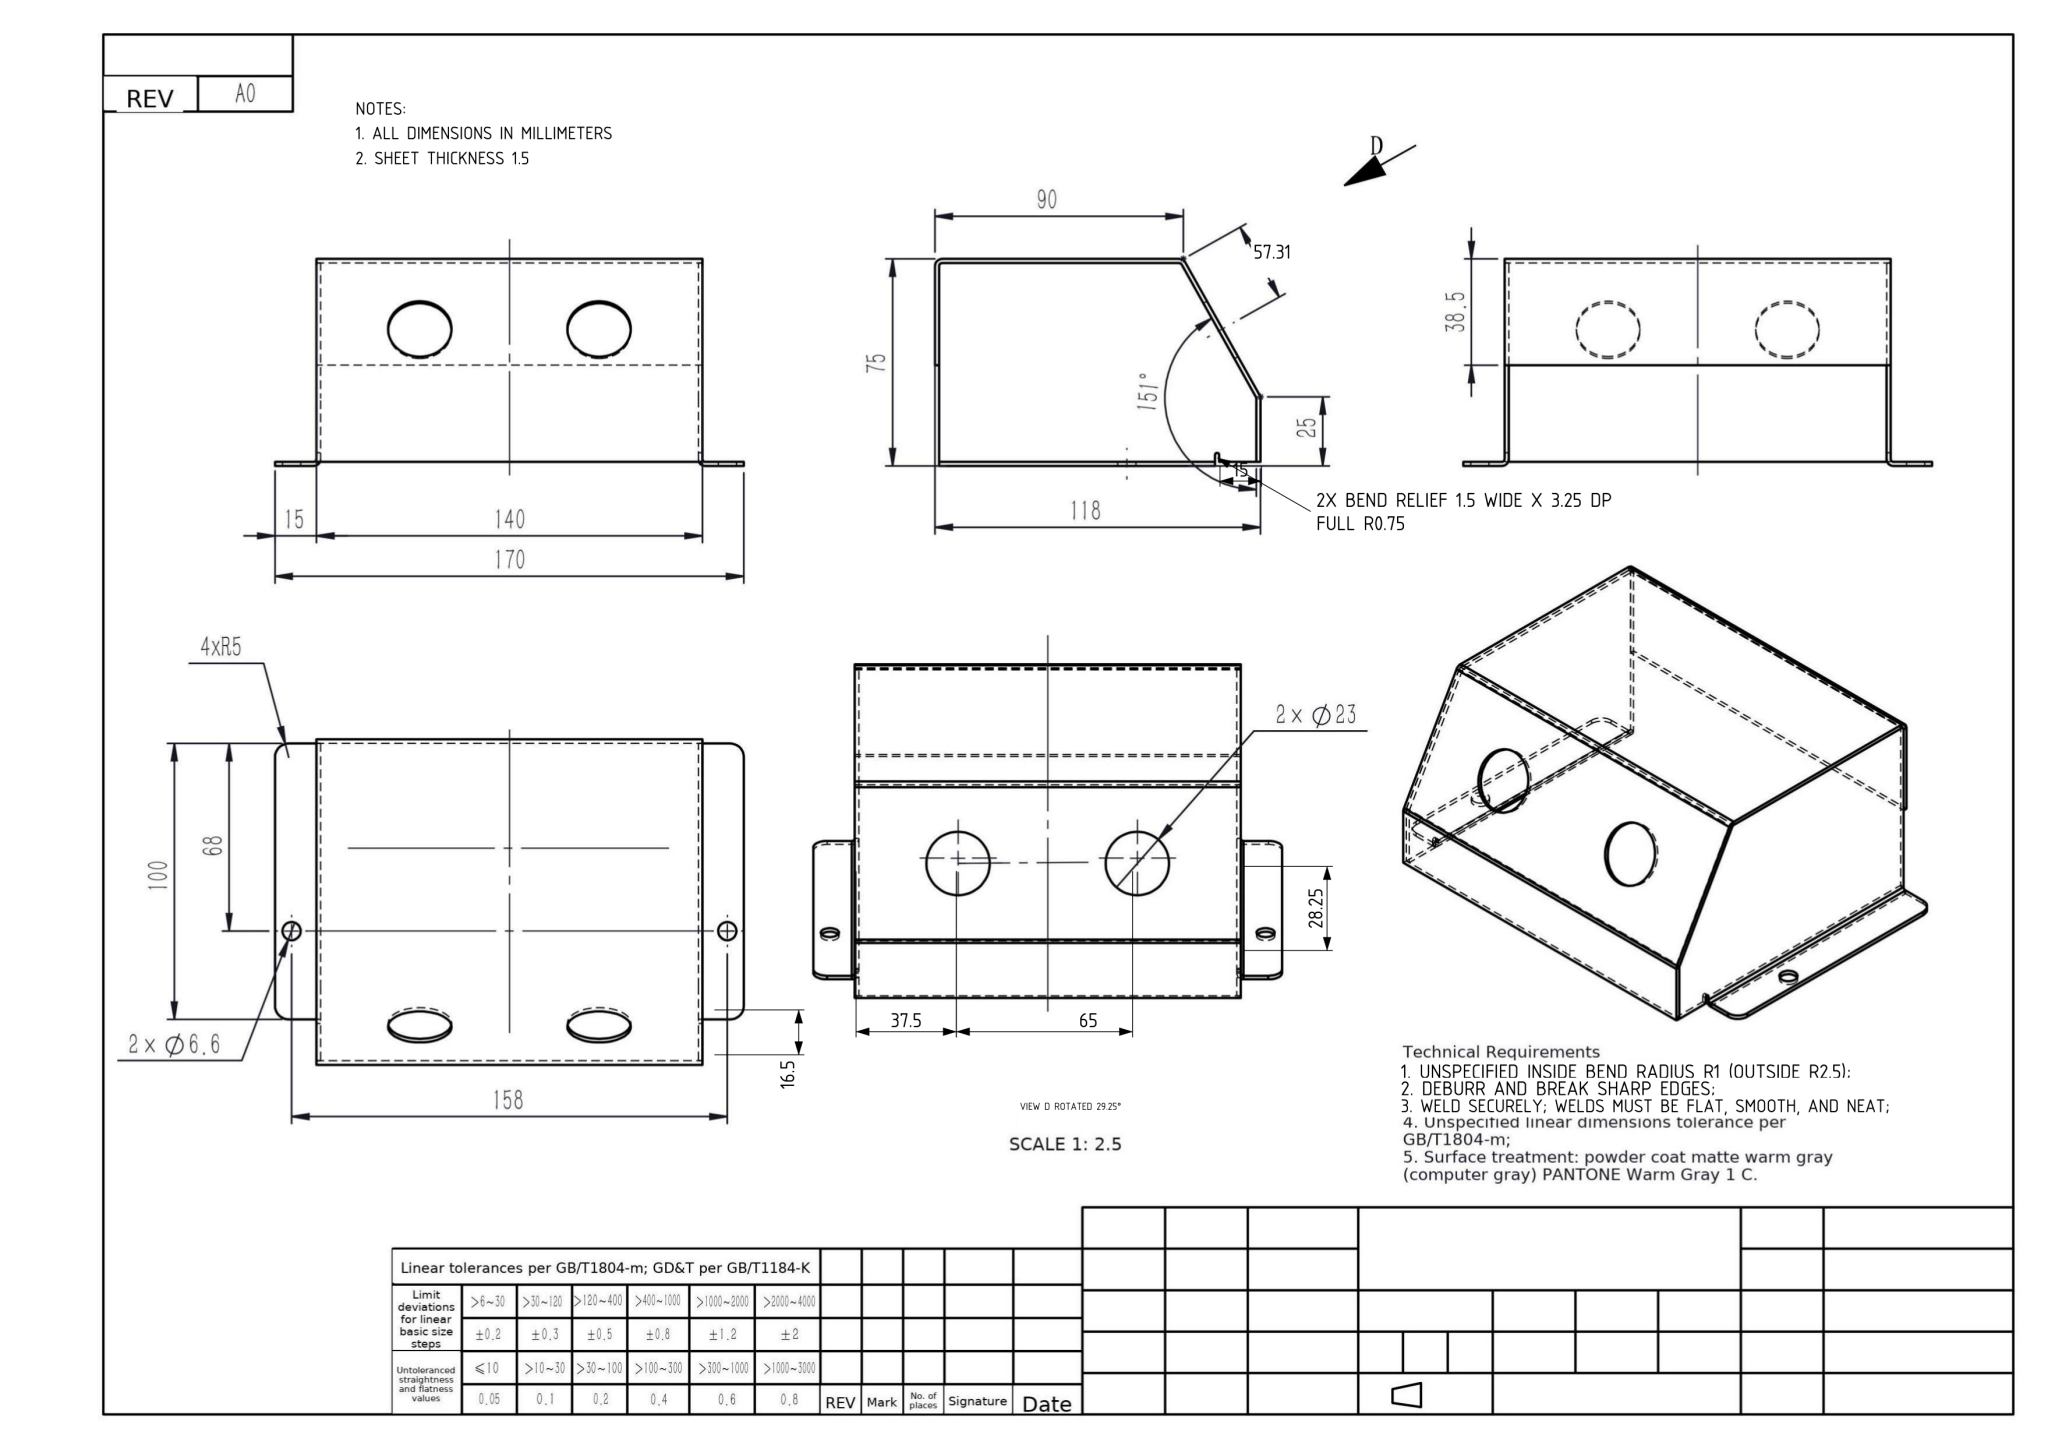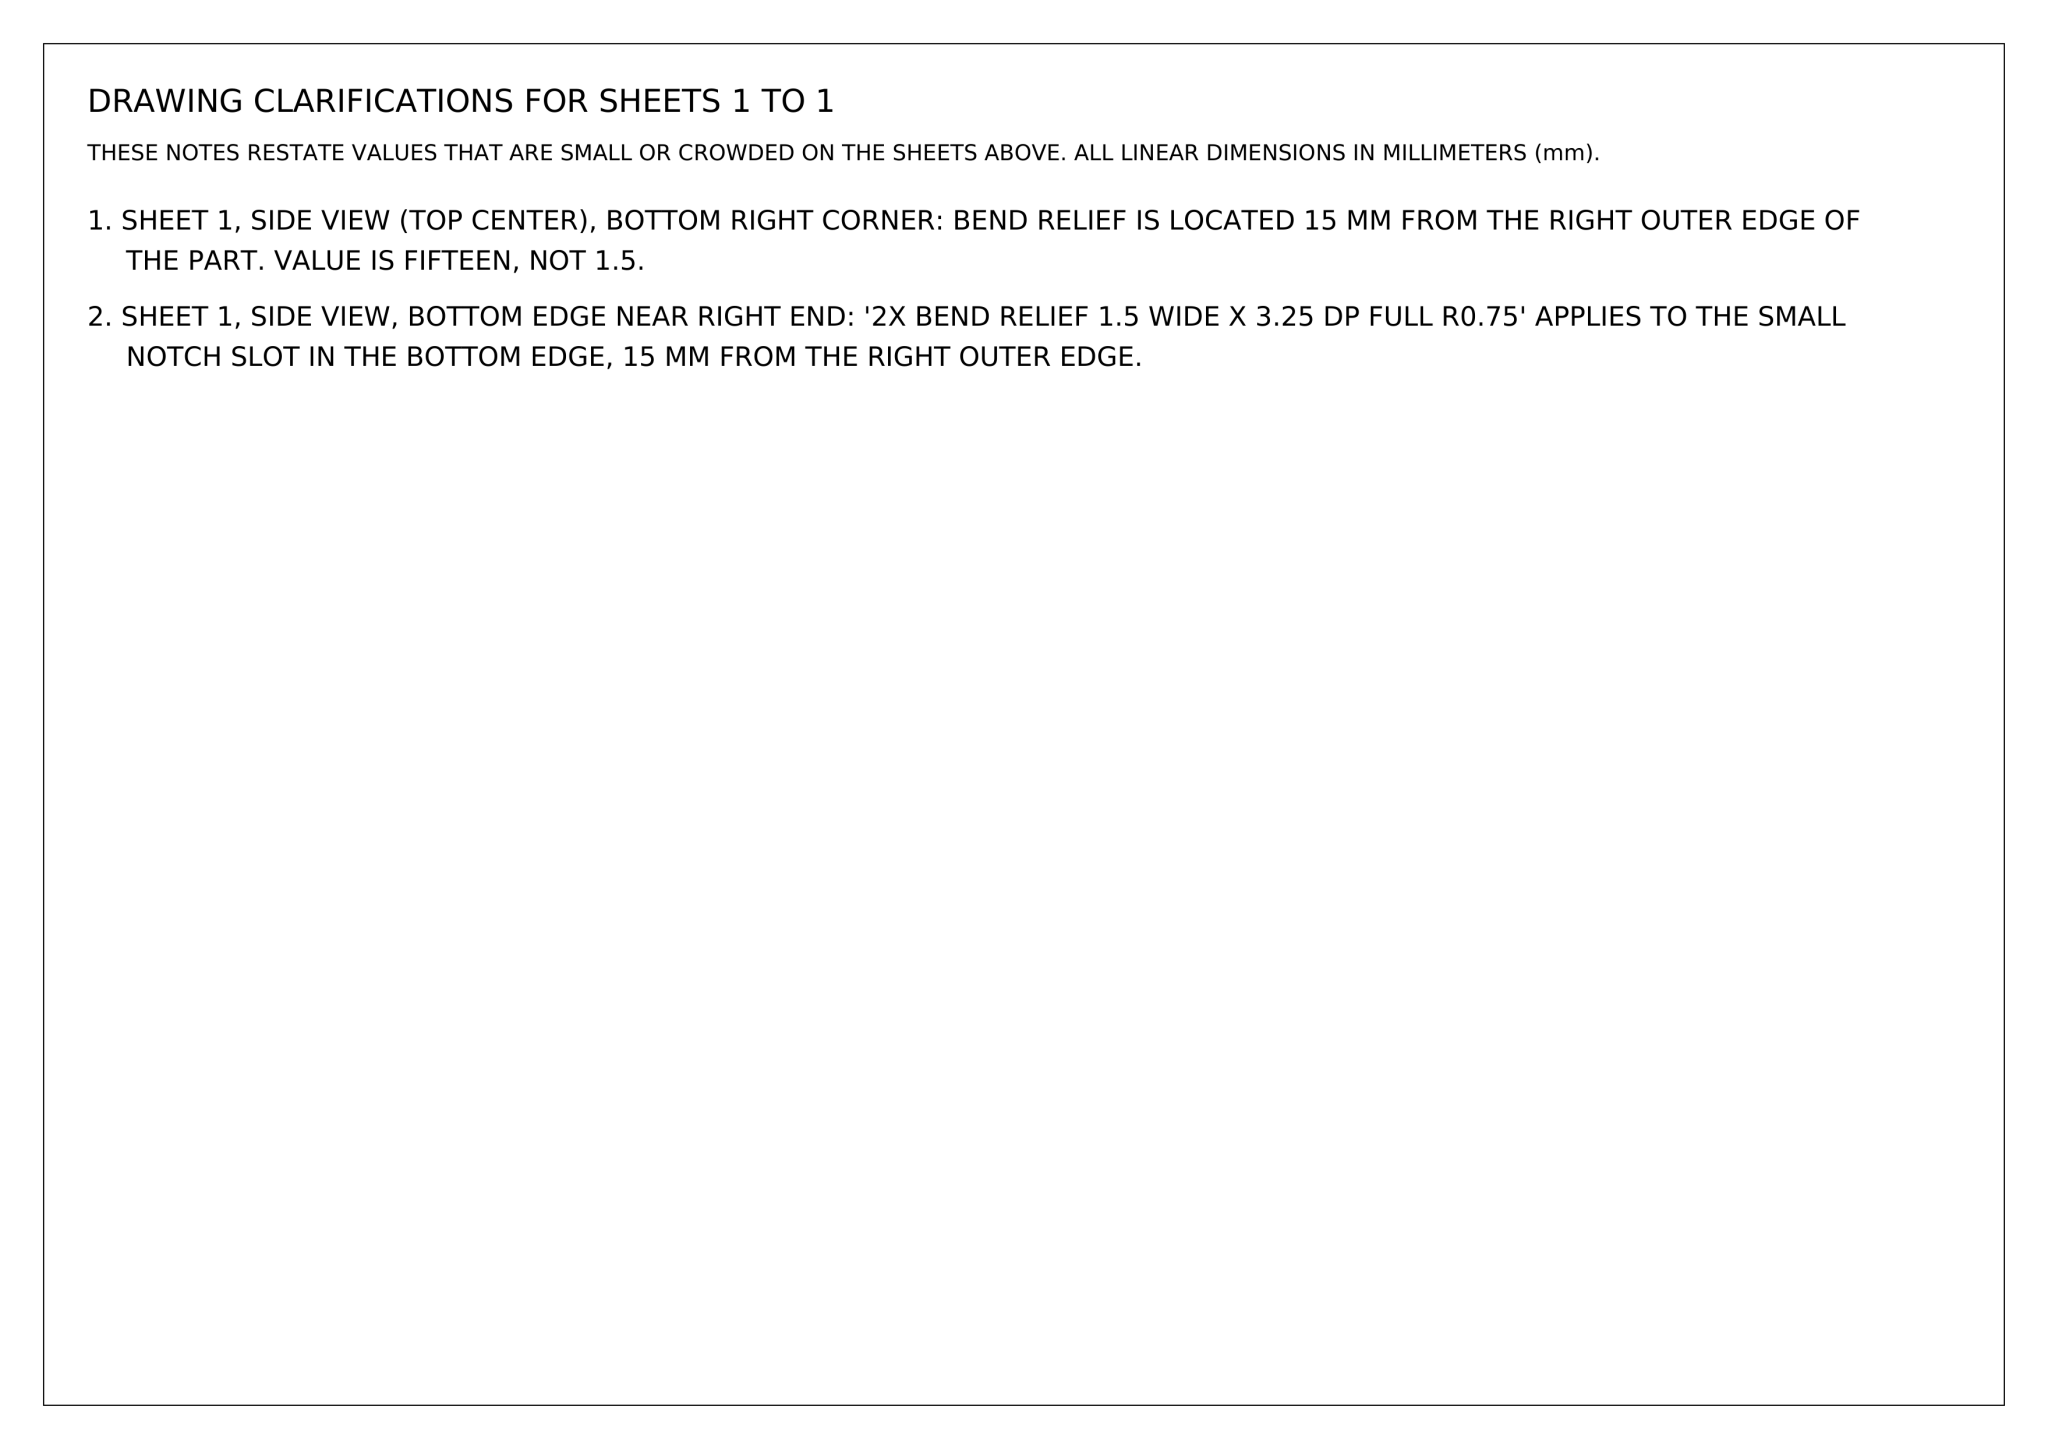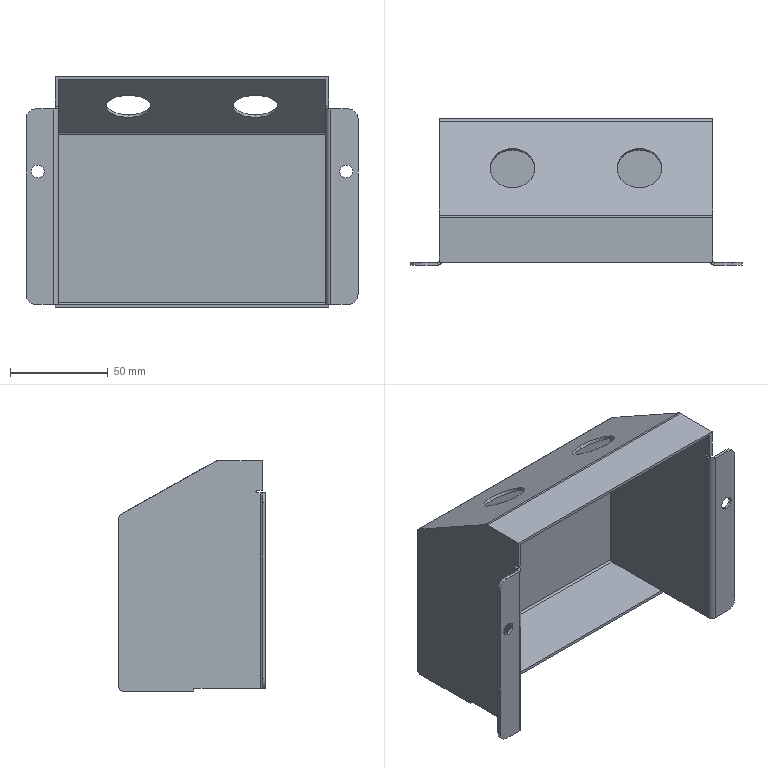Part | NX | mm | Dual-Oval Bore Stepped Bracket | 1 solid | 58 faces | box 170 x 75 x 118 mm | volume 69330 mm3 | plane 34 | cylinder 24 | commonest cylinder face diameters 2 x5 5 x5 10 x4 6.6 x4 23 x4 1.5 x2